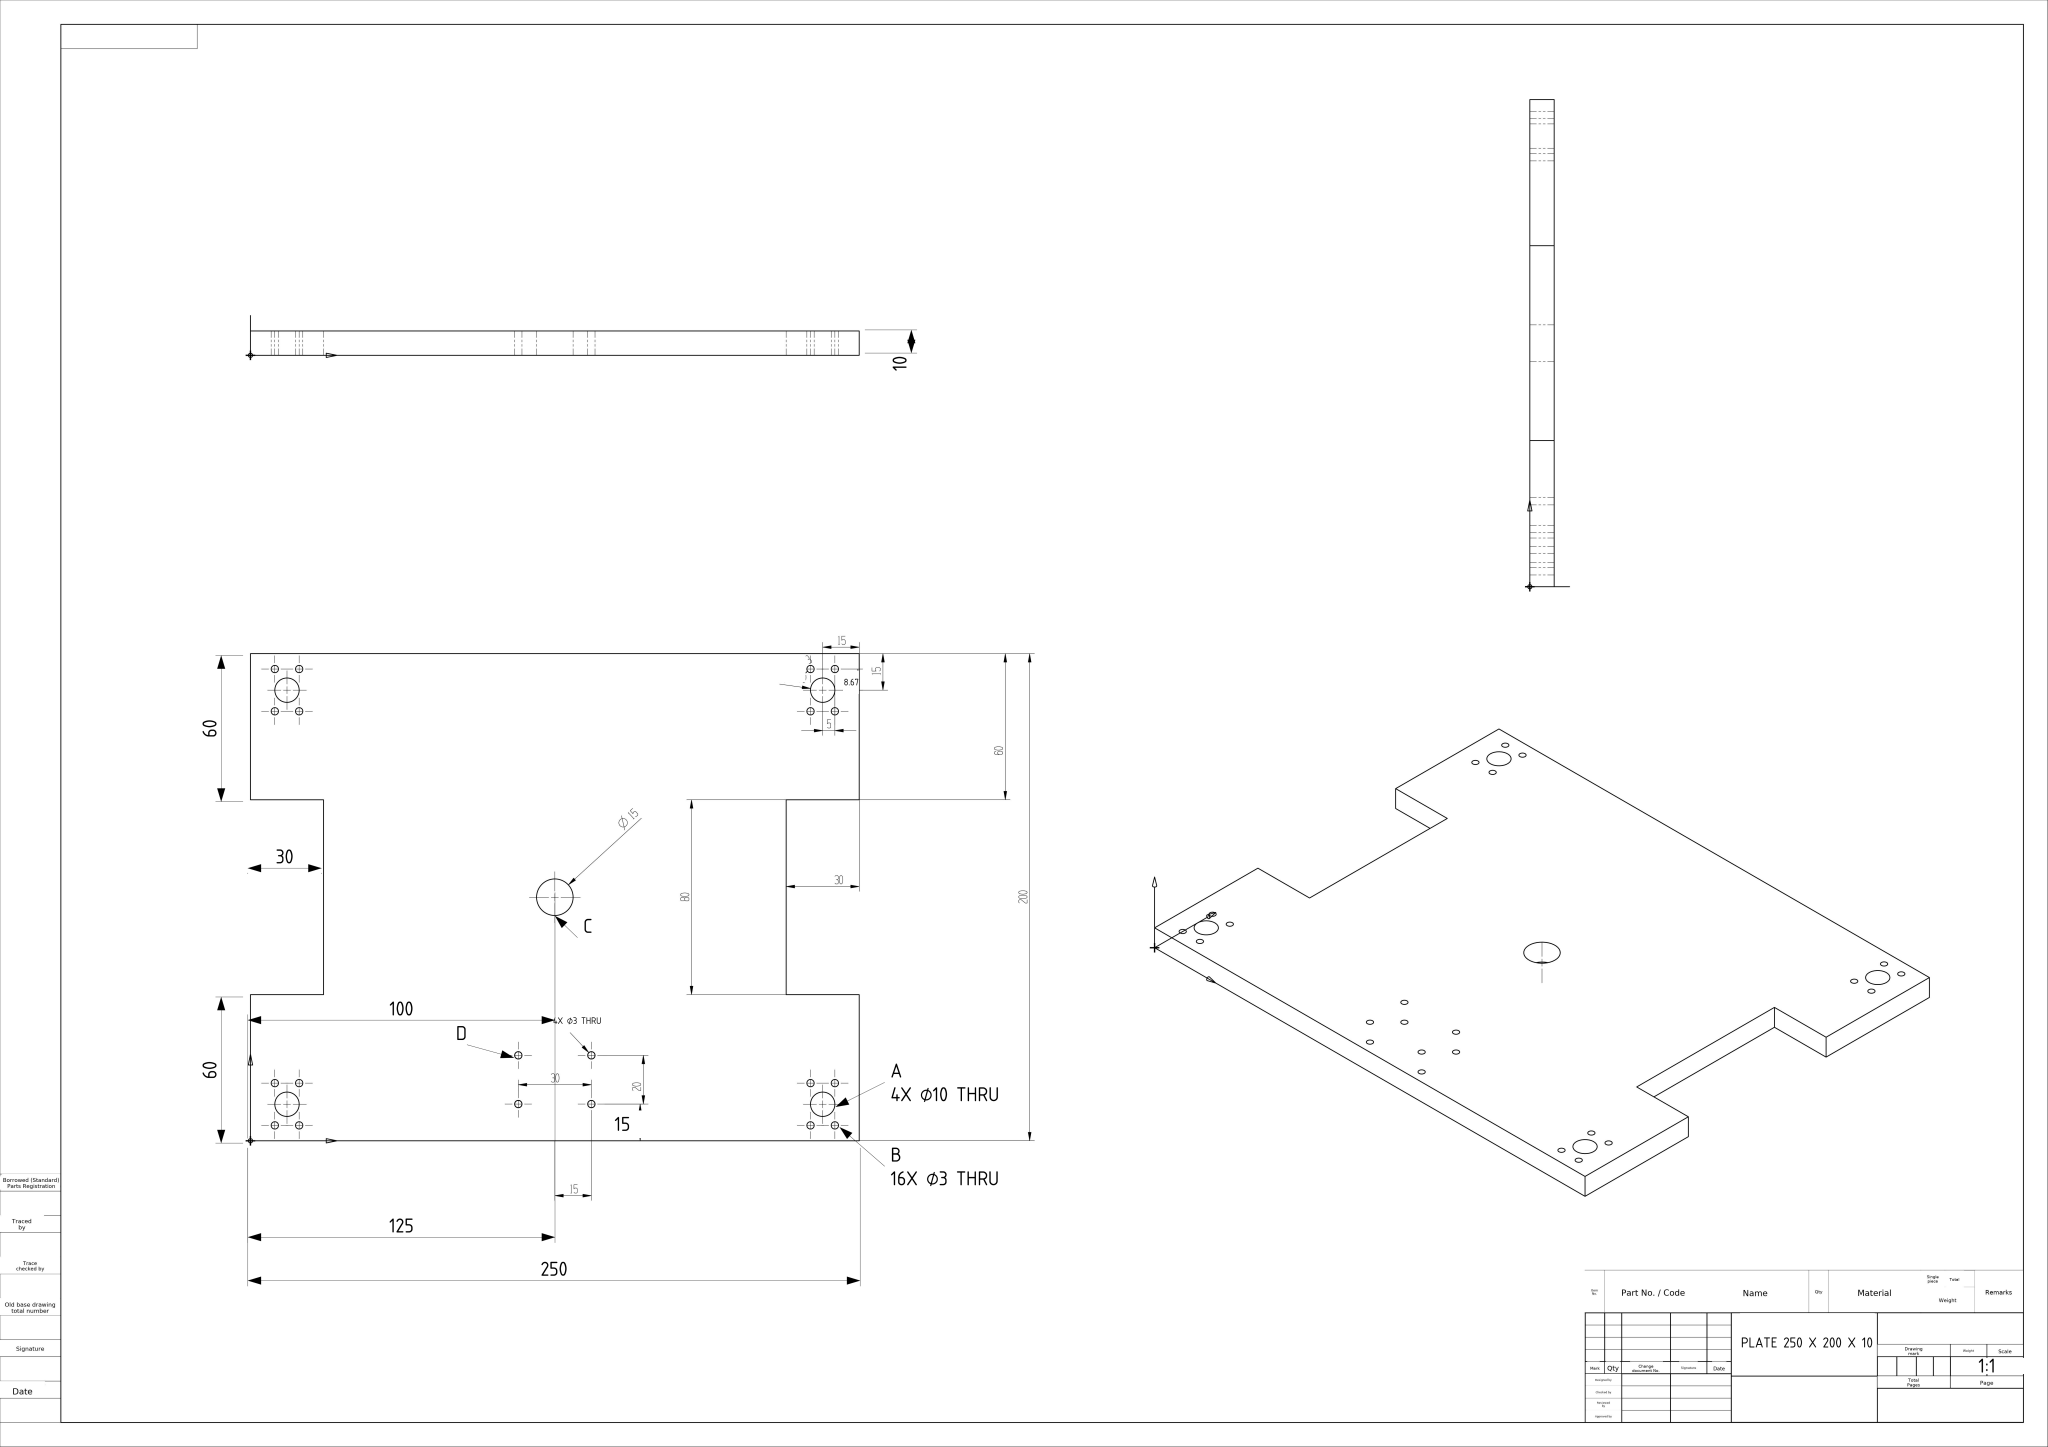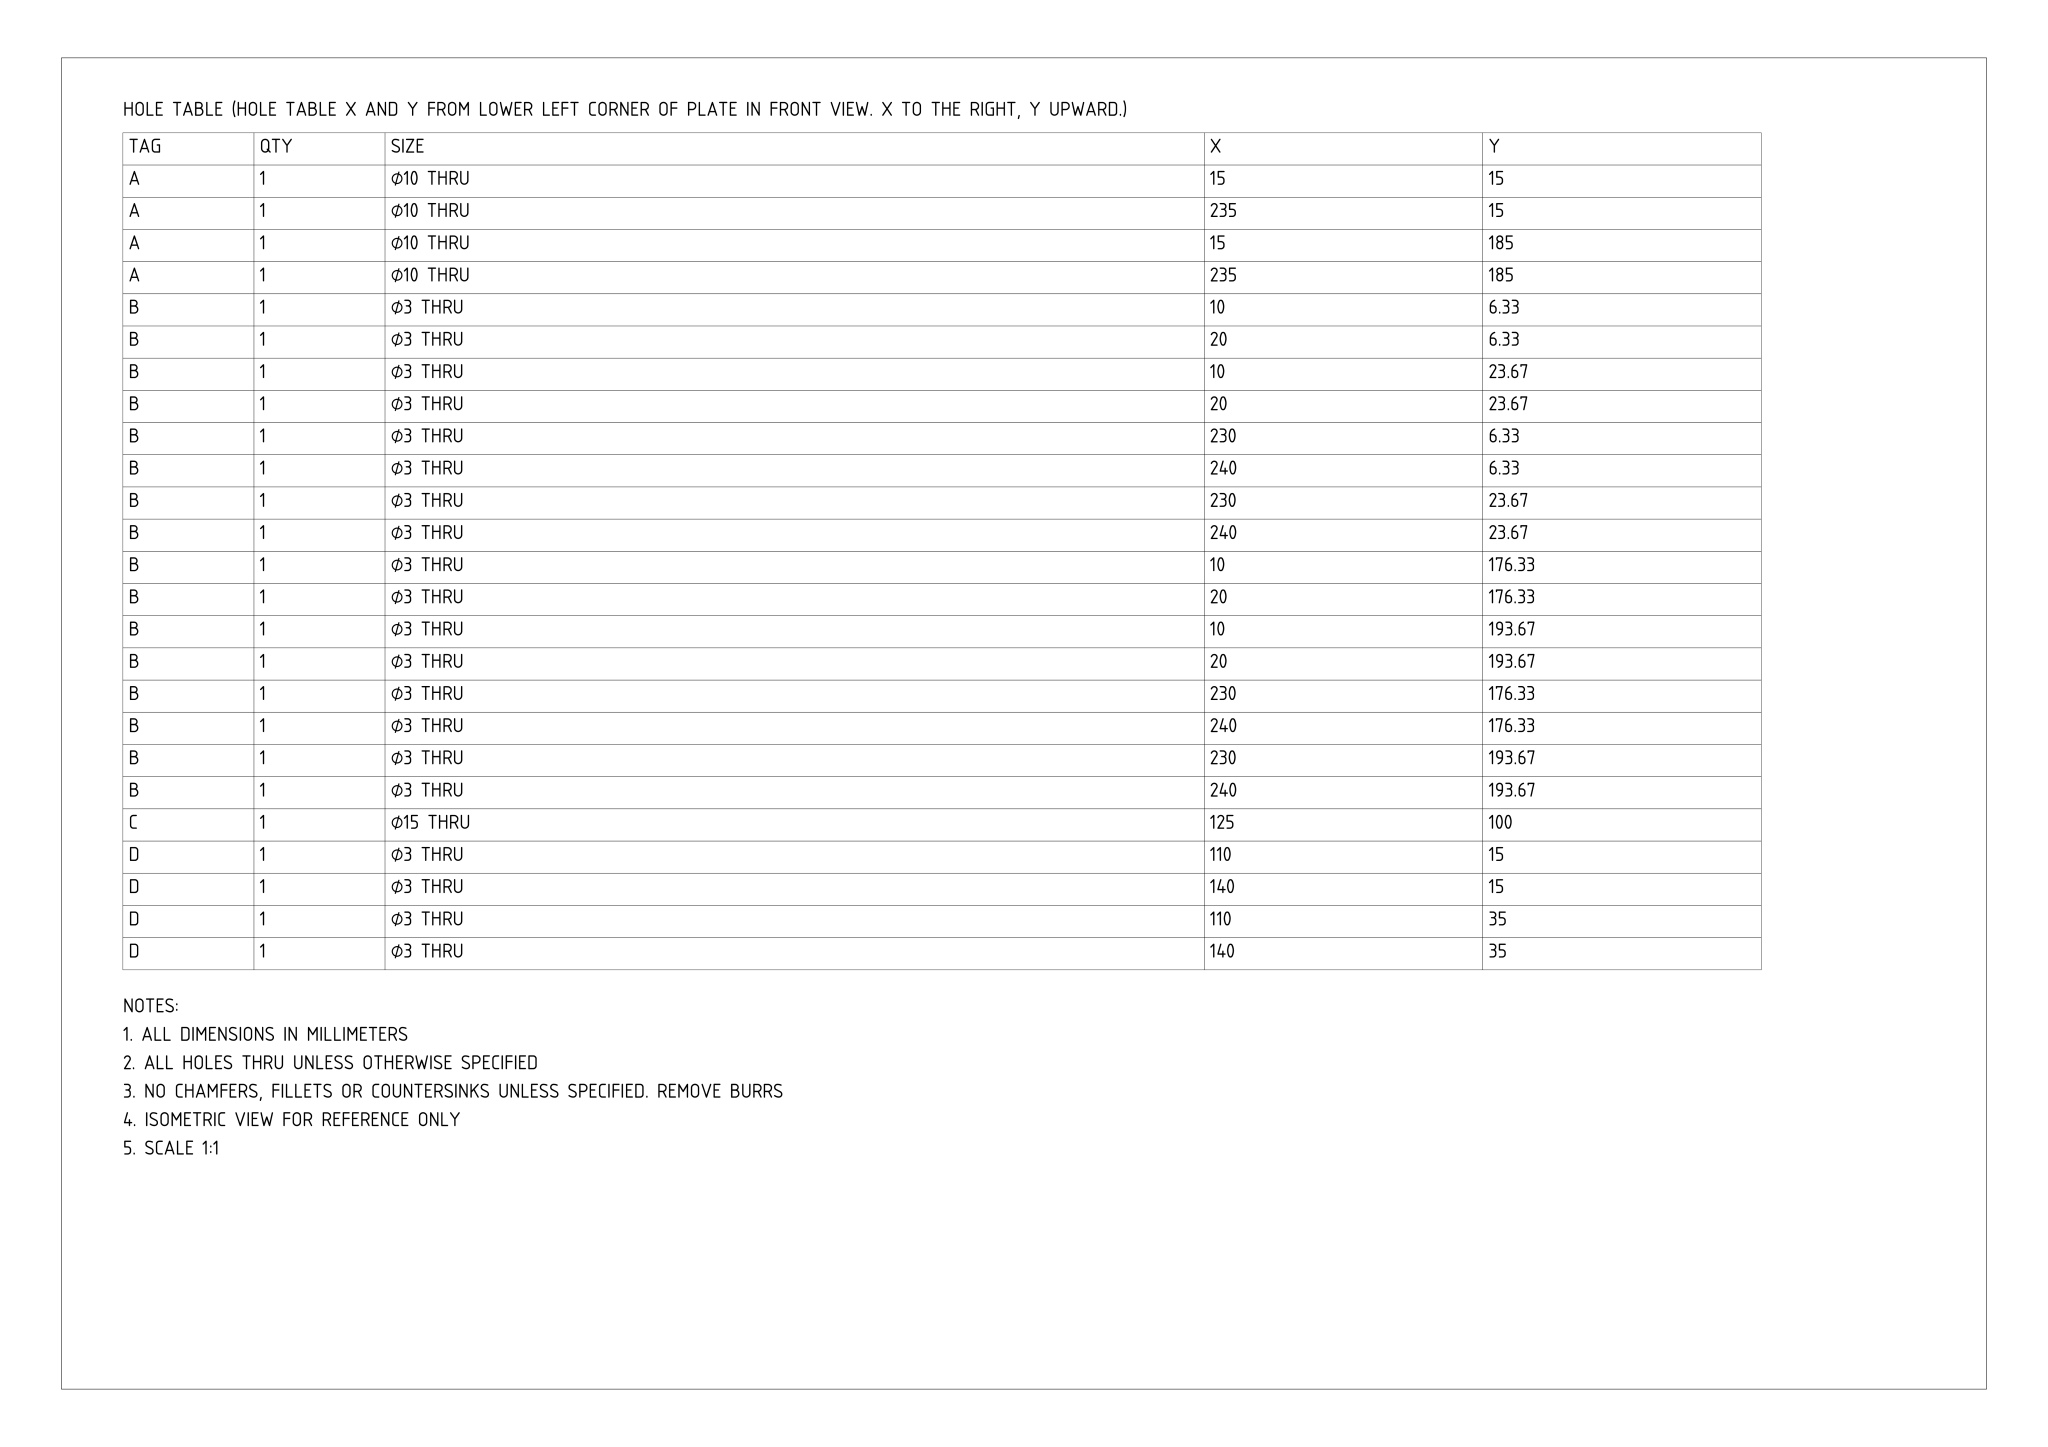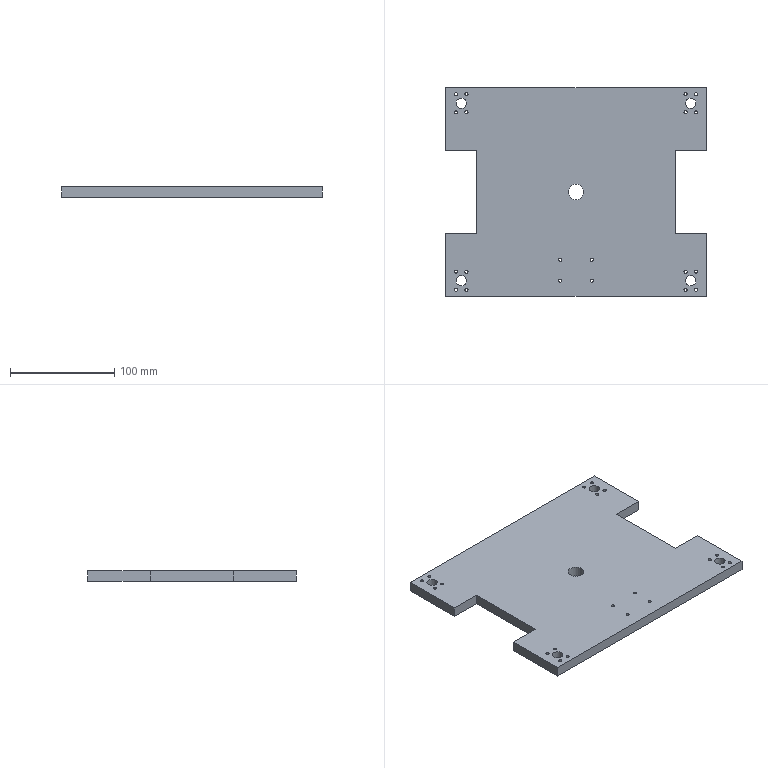Part | NX | mm | 1 solid | 39 faces | box 250 x 200 x 10 mm | volume 445678 mm3 | cylinder 25 | plane 14 | commonest cylinder face diameters 3 x20 10 x4 15 x1